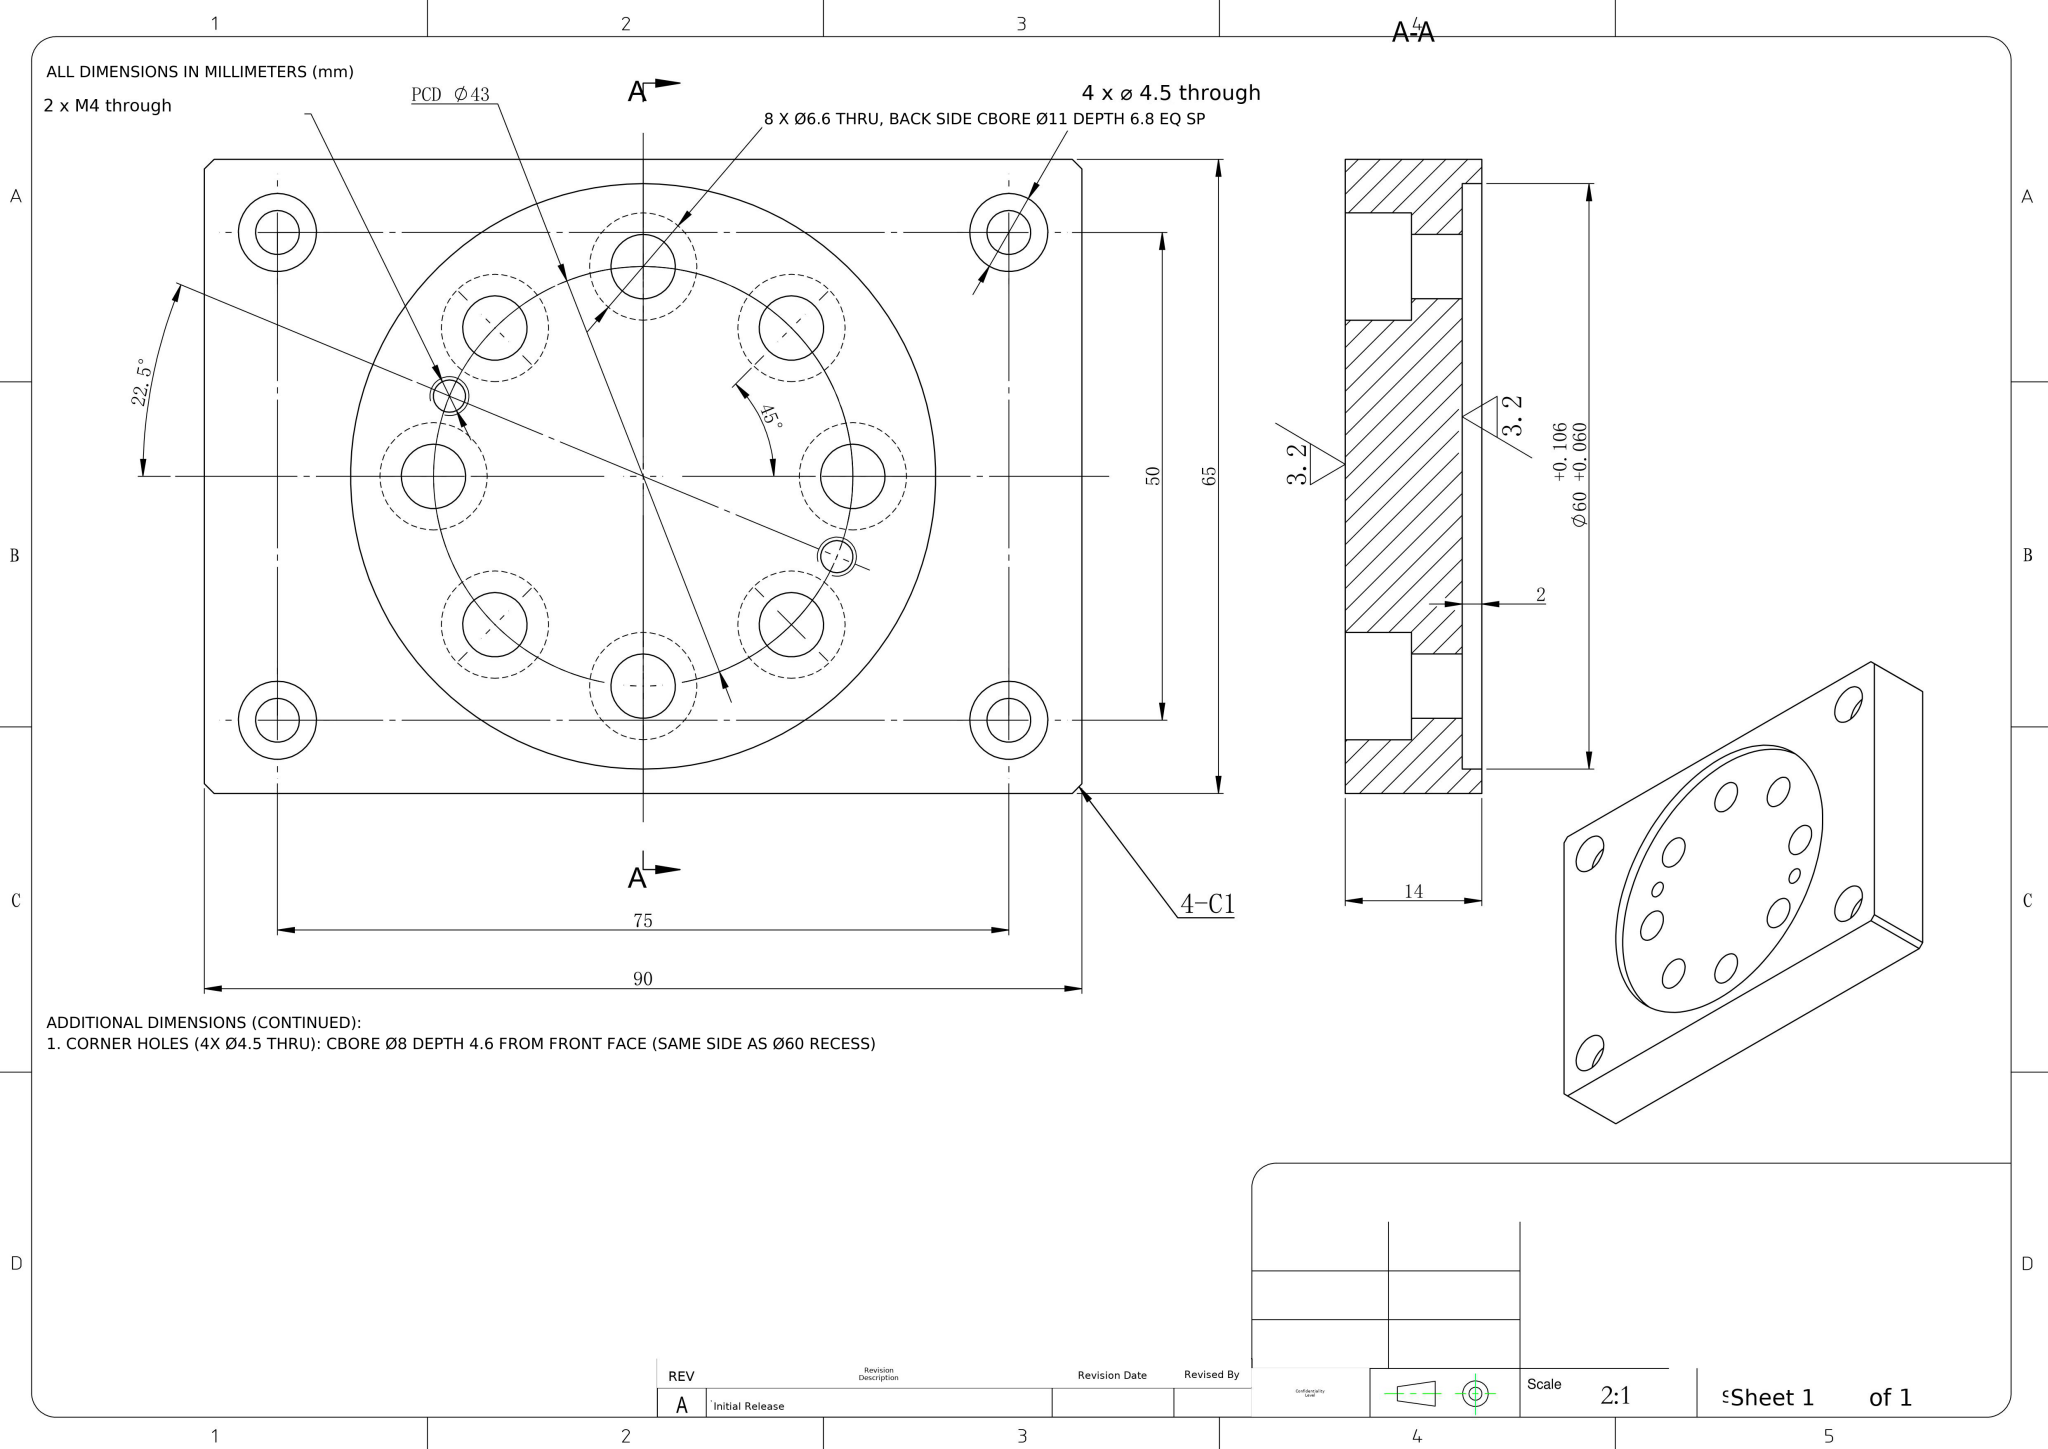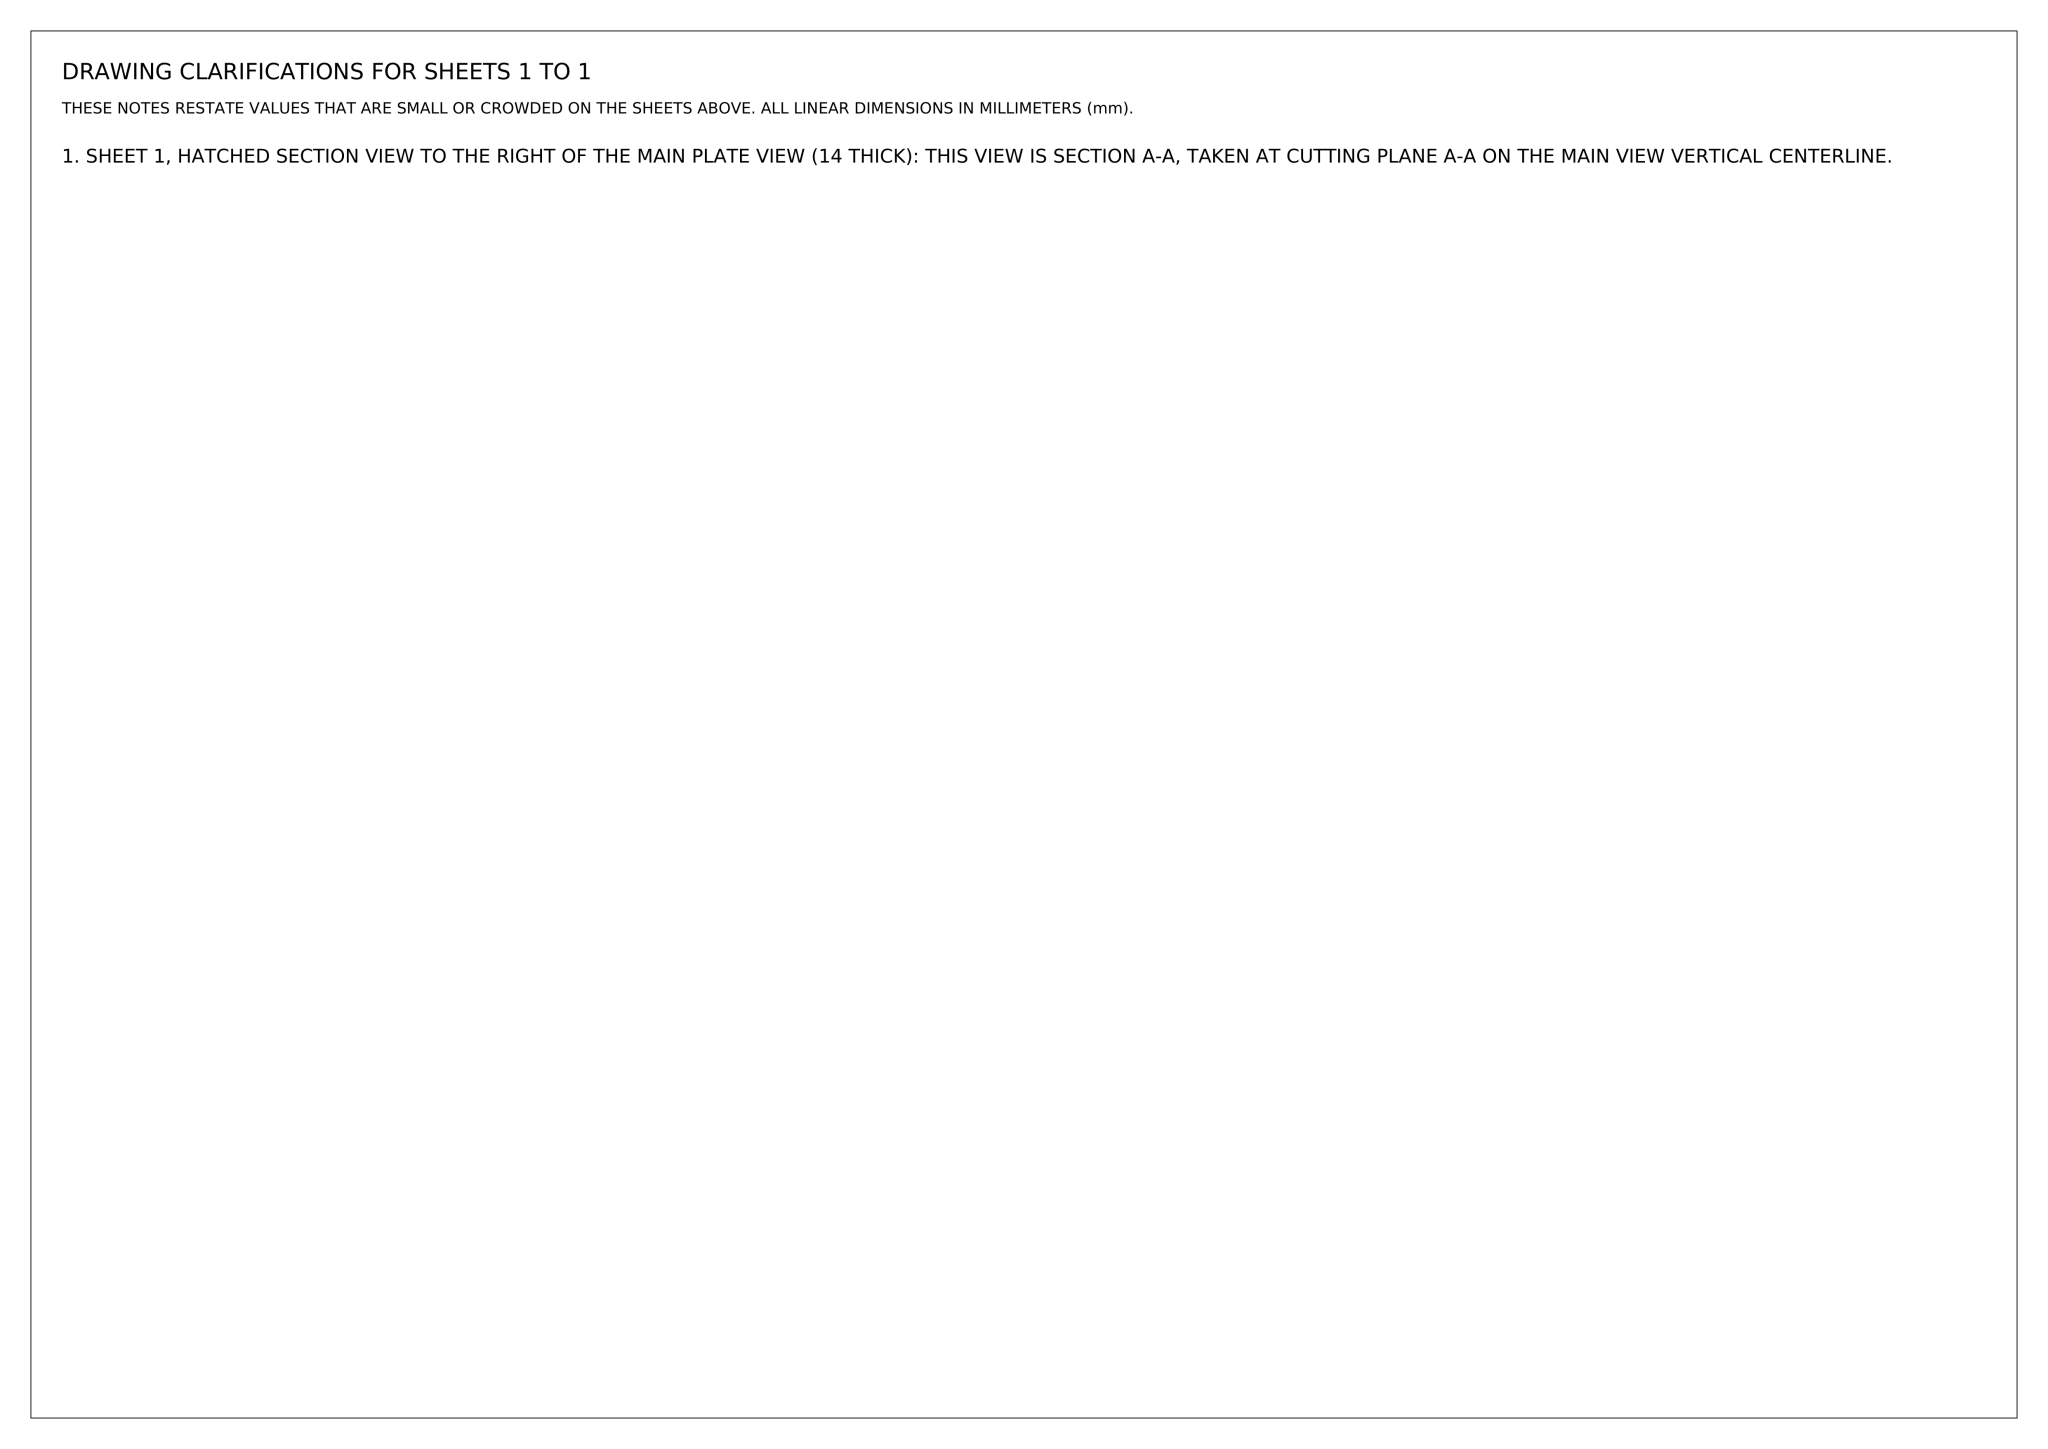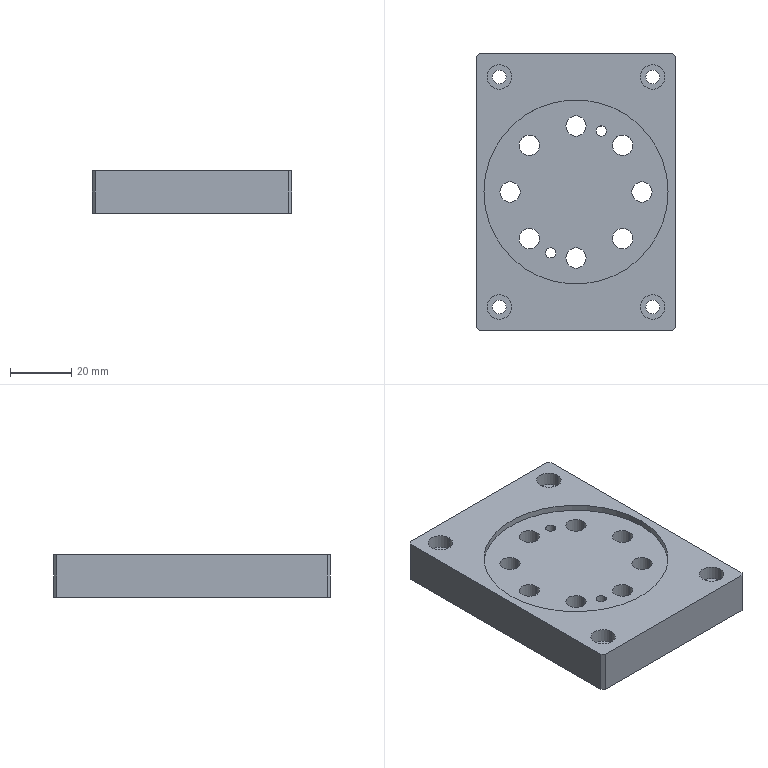Part | NX | mm | 1 solid | 77 faces | box 65 x 90 x 14 mm | volume 67896 mm3 | cylinder 54 | plane 23 | commonest cylinder face diameters 11 x16 6.6 x16 8 x8 4.5 x8 3.3 x4 60 x2